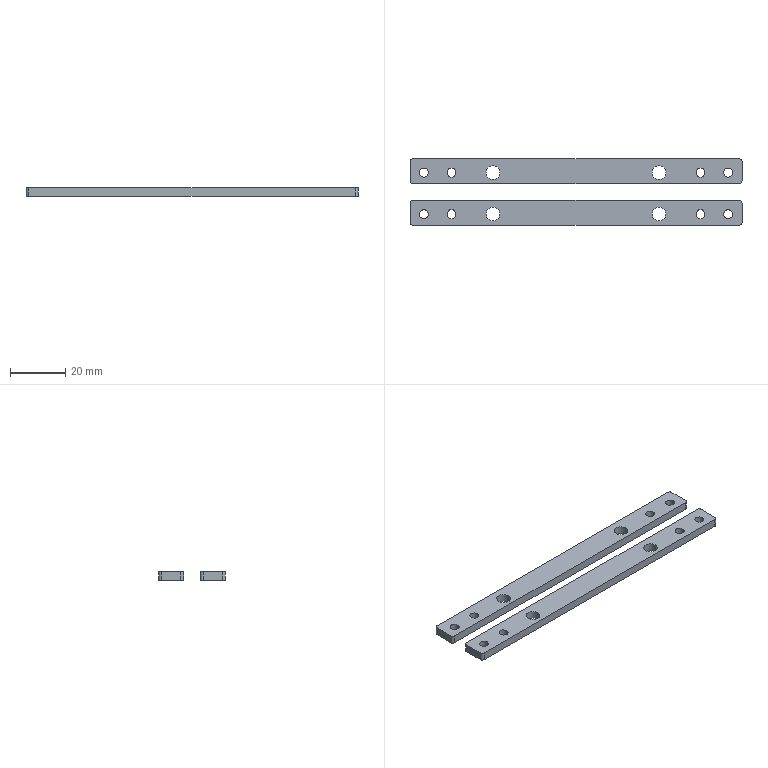CAM job | Mastercam | mm | 4 operations | part box 120 x 24 x 3
1. Contour (Ramp) | 3 - 3 平铣刀
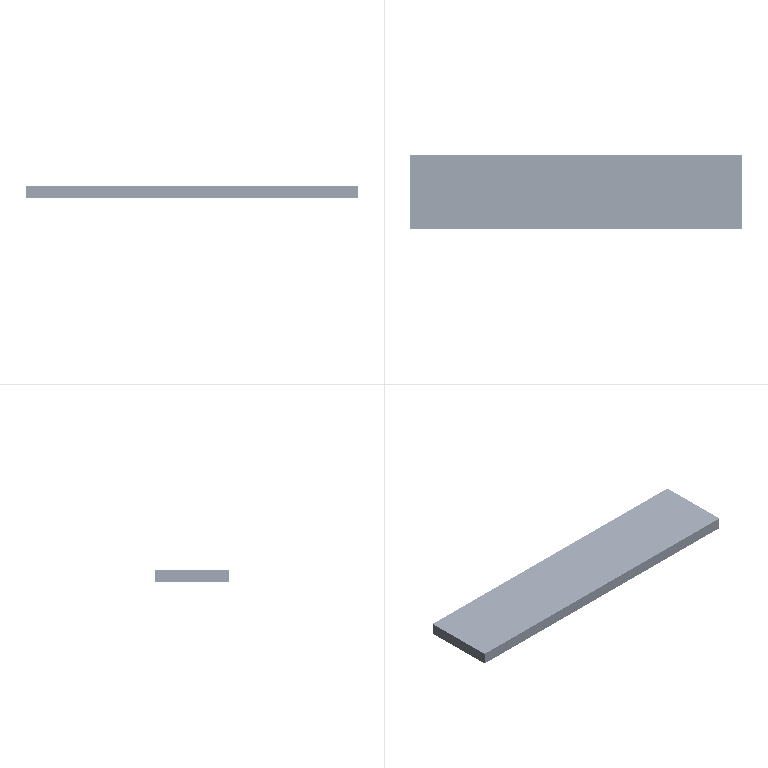2. Contour (2D) | 3 - 3 平铣刀
3. Contour (2D chamfer) | 7 - 4 倒角刀
4. Drill/Counterbore | 7 - 4 倒角刀